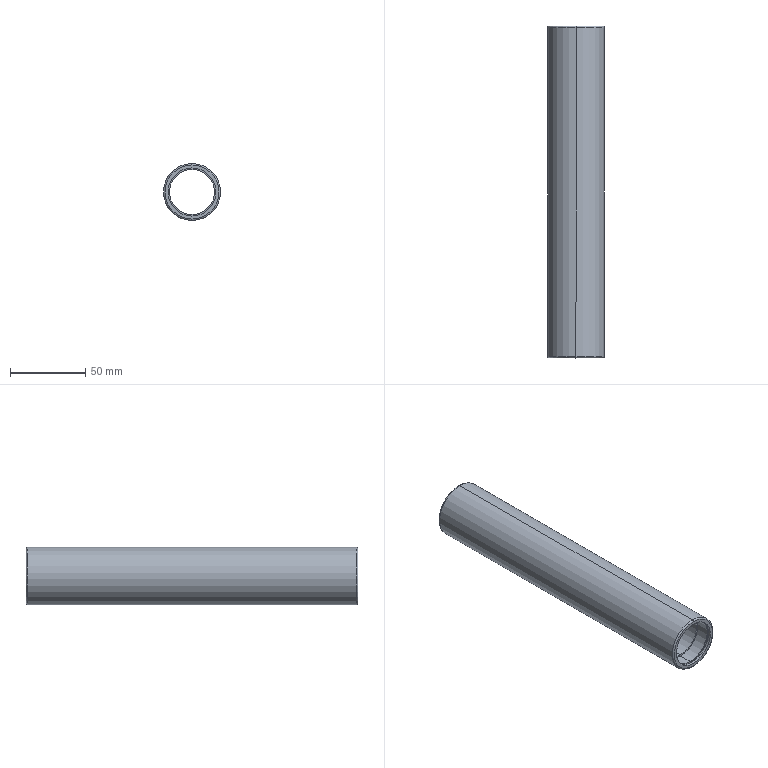Component | SolidWorks | 8TC-A15004-83-00-16_8TC-A15004-80-13A-1 | 1 solid | 28 faces | box 38 x 221 x 38 mm | volume 91799 mm3 | cylinder 16 | plane 8 | torus 4 | commonest cylinder face diameters 32 x8 33.7 x4 38 x2 30 x2 | material #45
build123d program:
from build123d import *

# Parameters (mm, degrees)
FILLET1_R = 1


with BuildPart() as part:
    # Sketch1 → Revolve1 (revolve)
    with BuildSketch(Plane(origin=(0, 0, 0), x_dir=(1, 0, 0), z_dir=(0, 1, 0)), mode=Mode.PRIVATE) as revolve1_sk:
        Polygon((98.5, 15), (-98.5, 15), (-98.5, 16), (-107.5, 16), (-107.5, 16.85), (-108.85, 16.85), (-108.85, 16), (-110.5, 16), (-110.5, 19), (110.5, 19), (110.5, 16), (108.85, 16), (108.85, 16.85), (107.5, 16.85), (107.5, 16), (98.5, 16), align=None)
    revolve(revolve1_sk.sketch.rotate(Axis((-29.776, 0, 0), (1, 0, 0)), 180), axis=Axis((-29.776, 0, 0), (1, 0, 0)))

    # Fillet1
    fillet1_edges = [part.edges().sort_by_distance(p)[0] for p in [
        (-110.5, 0, -19),
        (110.5, 0, -19),
    ]]
    fillet(fillet1_edges, radius=FILLET1_R)


solid = part.part

# Placed as in the assembly
solid = solid.moved(Location((40, 130, 60), (0, 0, 90)))
STEP:
#1=COLOUR_RGB('',0.7922,0.8196,0.9333);
#2=FILL_AREA_STYLE_COLOUR('',#1);
#3=FILL_AREA_STYLE('',(#2));
#4=SURFACE_STYLE_FILL_AREA(#3);
#5=SURFACE_SIDE_STYLE('',(#4));
#6=SURFACE_STYLE_USAGE(.BOTH.,#5);
#7=PRESENTATION_STYLE_ASSIGNMENT((#6));
#8=CARTESIAN_POINT('',(1.575,0.7677,3.071));
#9=VERTEX_POINT('',#8);
#10=CARTESIAN_POINT('',(1.575,0.7677,1.654));
#11=VERTEX_POINT('',#10);
#12=CARTESIAN_POINT('',(1.575,0.7677,2.362));
#13=DIRECTION('',(-0.,-1.,0.));
#14=DIRECTION('',(0.,0.,-1.));
#15=AXIS2_PLACEMENT_3D('',#12,#13,#14);
#16=CIRCLE('',#15,0.7087);
#17=EDGE_CURVE('',#9,#11,#16,.T.);
#18=ORIENTED_EDGE('',*,*,#17,.F.);
#19=CARTESIAN_POINT('',(1.575,0.8071,3.11));
#20=VERTEX_POINT('',#19);
#21=CARTESIAN_POINT('',(1.575,0.8071,3.071));
#22=DIRECTION('',(-1.,0.,-0.));
#23=DIRECTION('',(0.,-1.,0.));
#24=AXIS2_PLACEMENT_3D('',#21,#22,#23);
#25=CIRCLE('',#24,0.03937);
#26=EDGE_CURVE('',#9,#20,#25,.T.);
#27=ORIENTED_EDGE('',*,*,#26,.T.);
#28=CARTESIAN_POINT('',(1.575,0.8071,1.614));
#29=VERTEX_POINT('',#28);
#30=CARTESIAN_POINT('',(1.575,0.8071,2.362));
#31=DIRECTION('',(0.,1.,0.));
#32=DIRECTION('',(0.,0.,-1.));
#33=AXIS2_PLACEMENT_3D('',#30,#31,#32);
#34=CIRCLE('',#33,0.748);
#35=EDGE_CURVE('',#29,#20,#34,.T.);
#36=ORIENTED_EDGE('',*,*,#35,.F.);
#37=CARTESIAN_POINT('',(1.575,0.8071,1.654));
#38=DIRECTION('',(1.,-0.,0.));
#39=DIRECTION('',(0.,1.,0.));
#40=AXIS2_PLACEMENT_3D('',#37,#38,#39);
#41=CIRCLE('',#40,0.03937);
#42=EDGE_CURVE('',#11,#29,#41,.T.);
#43=ORIENTED_EDGE('',*,*,#42,.F.);
#44=EDGE_LOOP('',(#18,#27,#36,#43));
#45=FACE_OUTER_BOUND('',#44,.T.);
#46=CARTESIAN_POINT('',(1.575,0.8071,2.362));
#47=DIRECTION('',(0.,1.,0.));
#48=DIRECTION('',(0.,0.,-1.));
#49=AXIS2_PLACEMENT_3D('',#46,#47,#48);
#50=TOROIDAL_SURFACE('',#49,0.7087,0.03937);
#51=ADVANCED_FACE('',(#45),#50,.T.);
#52=CARTESIAN_POINT('',(1.575,9.469,1.654));
#53=VERTEX_POINT('',#52);
#54=CARTESIAN_POINT('',(1.575,9.469,3.071));
#55=VERTEX_POINT('',#54);
#56=CARTESIAN_POINT('',(1.575,9.469,2.362));
#57=DIRECTION('',(0.,1.,0.));
#58=DIRECTION('',(0.,0.,1.));
#59=AXIS2_PLACEMENT_3D('',#56,#57,#58);
#60=CIRCLE('',#59,0.7087);
#61=EDGE_CURVE('',#53,#55,#60,.T.);
#62=ORIENTED_EDGE('',*,*,#61,.F.);
#63=CARTESIAN_POINT('',(1.575,9.429,1.614));
#64=VERTEX_POINT('',#63);
#65=CARTESIAN_POINT('',(1.575,9.429,1.654));
#66=DIRECTION('',(-1.,0.,0.));
#67=DIRECTION('',(0.,-1.,0.));
#68=AXIS2_PLACEMENT_3D('',#65,#66,#67);
#69=CIRCLE('',#68,0.03937);
#70=EDGE_CURVE('',#53,#64,#69,.T.);
#71=ORIENTED_EDGE('',*,*,#70,.T.);
#72=CARTESIAN_POINT('',(1.575,9.429,3.11));
#73=VERTEX_POINT('',#72);
#74=CARTESIAN_POINT('',(1.575,9.429,2.362));
#75=DIRECTION('',(-0.,-1.,0.));
#76=DIRECTION('',(0.,0.,1.));
#77=AXIS2_PLACEMENT_3D('',#74,#75,#76);
#78=CIRCLE('',#77,0.748);
#79=EDGE_CURVE('',#73,#64,#78,.T.);
#80=ORIENTED_EDGE('',*,*,#79,.F.);
#81=CARTESIAN_POINT('',(1.575,9.429,3.071));
#82=DIRECTION('',(1.,-0.,0.));
#83=DIRECTION('',(0.,1.,0.));
#84=AXIS2_PLACEMENT_3D('',#81,#82,#83);
#85=CIRCLE('',#84,0.03937);
#86=EDGE_CURVE('',#55,#73,#85,.T.);
#87=ORIENTED_EDGE('',*,*,#86,.F.);
#88=EDGE_LOOP('',(#62,#71,#80,#87));
#89=FACE_OUTER_BOUND('',#88,.T.);
#90=CARTESIAN_POINT('',(1.575,9.429,2.362));
#91=DIRECTION('',(-0.,-1.,0.));
#92=DIRECTION('',(0.,0.,1.));
#93=AXIS2_PLACEMENT_3D('',#90,#91,#92);
#94=TOROIDAL_SURFACE('',#93,0.7087,0.03937);
#95=ADVANCED_FACE('',(#89),#94,.T.);
#96=CARTESIAN_POINT('',(1.575,1.24,1.732));
#97=VERTEX_POINT('',#96);
#98=CARTESIAN_POINT('',(1.575,1.24,2.992));
#99=VERTEX_POINT('',#98);
#100=CARTESIAN_POINT('',(1.575,1.24,2.362));
#101=DIRECTION('',(-0.,-1.,0.));
#102=DIRECTION('',(0.,0.,1.));
#103=AXIS2_PLACEMENT_3D('',#100,#101,#102);
#104=CIRCLE('',#103,0.6299);
#105=EDGE_CURVE('',#97,#99,#104,.T.);
#106=ORIENTED_EDGE('',*,*,#105,.F.);
#107=CARTESIAN_POINT('',(1.575,0.8858,1.732));
#108=VERTEX_POINT('',#107);
#109=CARTESIAN_POINT('',(1.575,3.946,1.732));
#110=DIRECTION('',(-0.,-1.,0.));
#111=VECTOR('',#110,39.37);
#112=LINE('',#109,#111);
#113=EDGE_CURVE('',#97,#108,#112,.T.);
#114=ORIENTED_EDGE('',*,*,#113,.T.);
#115=CARTESIAN_POINT('',(1.575,0.8858,2.992));
#116=VERTEX_POINT('',#115);
#117=CARTESIAN_POINT('',(1.575,0.8858,2.362));
#118=DIRECTION('',(-0.,-1.,0.));
#119=DIRECTION('',(0.,0.,1.));
#120=AXIS2_PLACEMENT_3D('',#117,#118,#119);
#121=CIRCLE('',#120,0.6299);
#122=EDGE_CURVE('',#108,#116,#121,.T.);
#123=ORIENTED_EDGE('',*,*,#122,.T.);
#124=CARTESIAN_POINT('',(1.575,3.946,2.992));
#125=DIRECTION('',(-0.,-1.,0.));
#126=VECTOR('',#125,39.37);
#127=LINE('',#124,#126);
#128=EDGE_CURVE('',#99,#116,#127,.T.);
#129=ORIENTED_EDGE('',*,*,#128,.F.);
#130=EDGE_LOOP('',(#106,#114,#123,#129));
#131=FACE_OUTER_BOUND('',#130,.T.);
#132=CARTESIAN_POINT('',(1.575,3.946,2.362));
#133=DIRECTION('',(-0.,-1.,0.));
#134=DIRECTION('',(0.,0.,1.));
#135=AXIS2_PLACEMENT_3D('',#132,#133,#134);
#136=CYLINDRICAL_SURFACE('',#135,0.6299);
#137=ADVANCED_FACE('',(#131),#136,.F.);
#138=CARTESIAN_POINT('',(1.575,0.8858,1.699));
#139=VERTEX_POINT('',#138);
#140=CARTESIAN_POINT('',(1.575,0.8858,3.026));
#141=VERTEX_POINT('',#140);
#142=CARTESIAN_POINT('',(1.575,0.8858,2.362));
#143=DIRECTION('',(-0.,-1.,0.));
#144=DIRECTION('',(0.,0.,1.));
#145=AXIS2_PLACEMENT_3D('',#142,#143,#144);
#146=CIRCLE('',#145,0.6634);
#147=EDGE_CURVE('',#139,#141,#146,.T.);
#148=ORIENTED_EDGE('',*,*,#147,.F.);
#149=CARTESIAN_POINT('',(1.575,0.8327,1.699));
#150=VERTEX_POINT('',#149);
#151=CARTESIAN_POINT('',(1.575,3.946,1.699));
#152=DIRECTION('',(-0.,-1.,0.));
#153=VECTOR('',#152,39.37);
#154=LINE('',#151,#153);
#155=EDGE_CURVE('',#139,#150,#154,.T.);
#156=ORIENTED_EDGE('',*,*,#155,.T.);
#157=CARTESIAN_POINT('',(1.575,0.8327,3.026));
#158=VERTEX_POINT('',#157);
#159=CARTESIAN_POINT('',(1.575,0.8327,2.362));
#160=DIRECTION('',(-0.,-1.,0.));
#161=DIRECTION('',(0.,0.,1.));
#162=AXIS2_PLACEMENT_3D('',#159,#160,#161);
#163=CIRCLE('',#162,0.6634);
#164=EDGE_CURVE('',#150,#158,#163,.T.);
#165=ORIENTED_EDGE('',*,*,#164,.T.);
#166=CARTESIAN_POINT('',(1.575,3.946,3.026));
#167=DIRECTION('',(-0.,-1.,0.));
#168=VECTOR('',#167,39.37);
#169=LINE('',#166,#168);
#170=EDGE_CURVE('',#141,#158,#169,.T.);
#171=ORIENTED_EDGE('',*,*,#170,.F.);
#172=EDGE_LOOP('',(#148,#156,#165,#171));
#173=FACE_OUTER_BOUND('',#172,.T.);
#174=CARTESIAN_POINT('',(1.575,3.946,2.362));
#175=DIRECTION('',(-0.,-1.,0.));
#176=DIRECTION('',(0.,0.,1.));
#177=AXIS2_PLACEMENT_3D('',#174,#175,#176);
#178=CYLINDRICAL_SURFACE('',#177,0.6634);
#179=ADVANCED_FACE('',(#173),#178,.F.);
#180=CARTESIAN_POINT('',(1.575,0.8327,1.732));
#181=VERTEX_POINT('',#180);
#182=CARTESIAN_POINT('',(1.575,0.8327,2.992));
#183=VERTEX_POINT('',#182);
#184=CARTESIAN_POINT('',(1.575,0.8327,2.362));
#185=DIRECTION('',(-0.,-1.,0.));
#186=DIRECTION('',(0.,0.,1.));
#187=AXIS2_PLACEMENT_3D('',#184,#185,#186);
#188=CIRCLE('',#187,0.6299);
#189=EDGE_CURVE('',#181,#183,#188,.T.);
#190=ORIENTED_EDGE('',*,*,#189,.F.);
#191=CARTESIAN_POINT('',(1.575,0.7677,1.732));
#192=VERTEX_POINT('',#191);
#193=CARTESIAN_POINT('',(1.575,3.946,1.732));
#194=DIRECTION('',(-0.,-1.,0.));
#195=VECTOR('',#194,39.37);
#196=LINE('',#193,#195);
#197=EDGE_CURVE('',#181,#192,#196,.T.);
#198=ORIENTED_EDGE('',*,*,#197,.T.);
#199=CARTESIAN_POINT('',(1.575,0.7677,2.992));
#200=VERTEX_POINT('',#199);
#201=CARTESIAN_POINT('',(1.575,0.7677,2.362));
#202=DIRECTION('',(-0.,-1.,0.));
#203=DIRECTION('',(0.,0.,1.));
#204=AXIS2_PLACEMENT_3D('',#201,#202,#203);
#205=CIRCLE('',#204,0.6299);
#206=EDGE_CURVE('',#192,#200,#205,.T.);
#207=ORIENTED_EDGE('',*,*,#206,.T.);
#208=CARTESIAN_POINT('',(1.575,3.946,2.992));
#209=DIRECTION('',(-0.,-1.,0.));
#210=VECTOR('',#209,39.37);
#211=LINE('',#208,#210);
#212=EDGE_CURVE('',#183,#200,#211,.T.);
#213=ORIENTED_EDGE('',*,*,#212,.F.);
#214=EDGE_LOOP('',(#190,#198,#207,#213));
#215=FACE_OUTER_BOUND('',#214,.T.);
#216=CARTESIAN_POINT('',(1.575,3.946,2.362));
#217=DIRECTION('',(-0.,-1.,0.));
#218=DIRECTION('',(0.,0.,1.));
#219=AXIS2_PLACEMENT_3D('',#216,#217,#218);
#220=CYLINDRICAL_SURFACE('',#219,0.6299);
#221=ADVANCED_FACE('',(#215),#220,.F.);
#222=ORIENTED_EDGE('',*,*,#79,.T.);
#223=CARTESIAN_POINT('',(1.575,3.946,1.614));
#224=DIRECTION('',(-0.,-1.,0.));
#225=VECTOR('',#224,39.37);
#226=LINE('',#223,#225);
#227=EDGE_CURVE('',#64,#29,#226,.T.);
#228=ORIENTED_EDGE('',*,*,#227,.T.);
#229=ORIENTED_EDGE('',*,*,#35,.T.);
#230=CARTESIAN_POINT('',(1.575,3.946,3.11));
#231=DIRECTION('',(-0.,-1.,0.));
#232=VECTOR('',#231,39.37);
#233=LINE('',#230,#232);
#234=EDGE_CURVE('',#73,#20,#233,.T.);
#235=ORIENTED_EDGE('',*,*,#234,.F.);
#236=EDGE_LOOP('',(#222,#228,#229,#235));
#237=FACE_OUTER_BOUND('',#236,.T.);
#238=CARTESIAN_POINT('',(1.575,3.946,2.362));
#239=DIRECTION('',(-0.,-1.,0.));
#240=DIRECTION('',(0.,0.,1.));
#241=AXIS2_PLACEMENT_3D('',#238,#239,#240);
#242=CYLINDRICAL_SURFACE('',#241,0.748);
#243=ADVANCED_FACE('',(#237),#242,.T.);
#244=CARTESIAN_POINT('',(1.575,9.469,1.732));
#245=VERTEX_POINT('',#244);
#246=CARTESIAN_POINT('',(1.575,9.469,2.992));
#247=VERTEX_POINT('',#246);
#248=CARTESIAN_POINT('',(1.575,9.469,2.362));
#249=DIRECTION('',(-0.,-1.,0.));
#250=DIRECTION('',(0.,0.,1.));
#251=AXIS2_PLACEMENT_3D('',#248,#249,#250);
#252=CIRCLE('',#251,0.6299);
#253=EDGE_CURVE('',#245,#247,#252,.T.);
#254=ORIENTED_EDGE('',*,*,#253,.F.);
#255=CARTESIAN_POINT('',(1.575,9.404,1.732));
#256=VERTEX_POINT('',#255);
#257=CARTESIAN_POINT('',(1.575,3.946,1.732));
#258=DIRECTION('',(-0.,-1.,0.));
#259=VECTOR('',#258,39.37);
#260=LINE('',#257,#259);
#261=EDGE_CURVE('',#245,#256,#260,.T.);
#262=ORIENTED_EDGE('',*,*,#261,.T.);
#263=CARTESIAN_POINT('',(1.575,9.404,2.992));
#264=VERTEX_POINT('',#263);
#265=CARTESIAN_POINT('',(1.575,9.404,2.362));
#266=DIRECTION('',(-0.,-1.,0.));
#267=DIRECTION('',(0.,0.,1.));
#268=AXIS2_PLACEMENT_3D('',#265,#266,#267);
#269=CIRCLE('',#268,0.6299);
#270=EDGE_CURVE('',#256,#264,#269,.T.);
#271=ORIENTED_EDGE('',*,*,#270,.T.);
#272=CARTESIAN_POINT('',(1.575,3.946,2.992));
#273=DIRECTION('',(-0.,-1.,0.));
#274=VECTOR('',#273,39.37);
#275=LINE('',#272,#274);
#276=EDGE_CURVE('',#247,#264,#275,.T.);
#277=ORIENTED_EDGE('',*,*,#276,.F.);
#278=EDGE_LOOP('',(#254,#262,#271,#277));
#279=FACE_OUTER_BOUND('',#278,.T.);
#280=CARTESIAN_POINT('',(1.575,3.946,2.362));
#281=DIRECTION('',(-0.,-1.,0.));
#282=DIRECTION('',(0.,0.,1.));
#283=AXIS2_PLACEMENT_3D('',#280,#281,#282);
#284=CYLINDRICAL_SURFACE('',#283,0.6299);
#285=ADVANCED_FACE('',(#279),#284,.F.);
#286=CARTESIAN_POINT('',(1.575,9.404,1.699));
#287=VERTEX_POINT('',#286);
#288=CARTESIAN_POINT('',(1.575,9.404,3.026));
#289=VERTEX_POINT('',#288);
#290=CARTESIAN_POINT('',(1.575,9.404,2.362));
#291=DIRECTION('',(-0.,-1.,0.));
#292=DIRECTION('',(0.,0.,1.));
#293=AXIS2_PLACEMENT_3D('',#290,#291,#292);
#294=CIRCLE('',#293,0.6634);
#295=EDGE_CURVE('',#287,#289,#294,.T.);
#296=ORIENTED_EDGE('',*,*,#295,.F.);
#297=CARTESIAN_POINT('',(1.575,9.35,1.699));
#298=VERTEX_POINT('',#297);
#299=CARTESIAN_POINT('',(1.575,3.946,1.699));
#300=DIRECTION('',(-0.,-1.,0.));
#301=VECTOR('',#300,39.37);
#302=LINE('',#299,#301);
#303=EDGE_CURVE('',#287,#298,#302,.T.);
#304=ORIENTED_EDGE('',*,*,#303,.T.);
#305=CARTESIAN_POINT('',(1.575,9.35,3.026));
#306=VERTEX_POINT('',#305);
#307=CARTESIAN_POINT('',(1.575,9.35,2.362));
#308=DIRECTION('',(-0.,-1.,0.));
#309=DIRECTION('',(0.,0.,1.));
#310=AXIS2_PLACEMENT_3D('',#307,#308,#309);
#311=CIRCLE('',#310,0.6634);
#312=EDGE_CURVE('',#298,#306,#311,.T.);
#313=ORIENTED_EDGE('',*,*,#312,.T.);
#314=CARTESIAN_POINT('',(1.575,3.946,3.026));
#315=DIRECTION('',(-0.,-1.,0.));
#316=VECTOR('',#315,39.37);
#317=LINE('',#314,#316);
#318=EDGE_CURVE('',#289,#306,#317,.T.);
#319=ORIENTED_EDGE('',*,*,#318,.F.);
#320=EDGE_LOOP('',(#296,#304,#313,#319));
#321=FACE_OUTER_BOUND('',#320,.T.);
#322=CARTESIAN_POINT('',(1.575,3.946,2.362));
#323=DIRECTION('',(-0.,-1.,0.));
#324=DIRECTION('',(0.,0.,1.));
#325=AXIS2_PLACEMENT_3D('',#322,#323,#324);
#326=CYLINDRICAL_SURFACE('',#325,0.6634);
#327=ADVANCED_FACE('',(#321),#326,.F.);
#328=CARTESIAN_POINT('',(1.575,9.35,1.732));
#329=VERTEX_POINT('',#328);
#330=CARTESIAN_POINT('',(1.575,9.35,2.992));
#331=VERTEX_POINT('',#330);
#332=CARTESIAN_POINT('',(1.575,9.35,2.362));
#333=DIRECTION('',(-0.,-1.,0.));
#334=DIRECTION('',(0.,0.,1.));
#335=AXIS2_PLACEMENT_3D('',#332,#333,#334);
#336=CIRCLE('',#335,0.6299);
#337=EDGE_CURVE('',#329,#331,#336,.T.);
#338=ORIENTED_EDGE('',*,*,#337,.F.);
#339=CARTESIAN_POINT('',(1.575,8.996,1.732));
#340=VERTEX_POINT('',#339);
#341=CARTESIAN_POINT('',(1.575,3.946,1.732));
#342=DIRECTION('',(-0.,-1.,0.));
#343=VECTOR('',#342,39.37);
#344=LINE('',#341,#343);
#345=EDGE_CURVE('',#329,#340,#344,.T.);
#346=ORIENTED_EDGE('',*,*,#345,.T.);
#347=CARTESIAN_POINT('',(1.575,8.996,2.992));
#348=VERTEX_POINT('',#347);
#349=CARTESIAN_POINT('',(1.575,8.996,2.362));
#350=DIRECTION('',(-0.,-1.,0.));
#351=DIRECTION('',(0.,0.,1.));
#352=AXIS2_PLACEMENT_3D('',#349,#350,#351);
#353=CIRCLE('',#352,0.6299);
#354=EDGE_CURVE('',#340,#348,#353,.T.);
#355=ORIENTED_EDGE('',*,*,#354,.T.);
#356=CARTESIAN_POINT('',(1.575,3.946,2.992));
#357=DIRECTION('',(-0.,-1.,0.));
#358=VECTOR('',#357,39.37);
#359=LINE('',#356,#358);
#360=EDGE_CURVE('',#331,#348,#359,.T.);
#361=ORIENTED_EDGE('',*,*,#360,.F.);
#362=EDGE_LOOP('',(#338,#346,#355,#361));
#363=FACE_OUTER_BOUND('',#362,.T.);
#364=CARTESIAN_POINT('',(1.575,3.946,2.362));
#365=DIRECTION('',(-0.,-1.,0.));
#366=DIRECTION('',(0.,0.,1.));
#367=AXIS2_PLACEMENT_3D('',#364,#365,#366);
#368=CYLINDRICAL_SURFACE('',#367,0.6299);
#369=ADVANCED_FACE('',(#363),#368,.F.);
#370=CARTESIAN_POINT('',(1.575,8.996,1.772));
#371=VERTEX_POINT('',#370);
#372=CARTESIAN_POINT('',(1.575,8.996,2.953));
#373=VERTEX_POINT('',#372);
#374=CARTESIAN_POINT('',(1.575,8.996,2.362));
#375=DIRECTION('',(-0.,-1.,0.));
#376=DIRECTION('',(0.,0.,1.));
#377=AXIS2_PLACEMENT_3D('',#374,#375,#376);
#378=CIRCLE('',#377,0.5906);
#379=EDGE_CURVE('',#371,#373,#378,.T.);
#380=ORIENTED_EDGE('',*,*,#379,.F.);
#381=CARTESIAN_POINT('',(1.575,1.24,1.772));
#382=VERTEX_POINT('',#381);
#383=CARTESIAN_POINT('',(1.575,3.946,1.772));
#384=DIRECTION('',(-0.,-1.,0.));
#385=VECTOR('',#384,39.37);
#386=LINE('',#383,#385);
#387=EDGE_CURVE('',#371,#382,#386,.T.);
#388=ORIENTED_EDGE('',*,*,#387,.T.);
#389=CARTESIAN_POINT('',(1.575,1.24,2.953));
#390=VERTEX_POINT('',#389);
#391=CARTESIAN_POINT('',(1.575,1.24,2.362));
#392=DIRECTION('',(-0.,-1.,0.));
#393=DIRECTION('',(0.,0.,1.));
#394=AXIS2_PLACEMENT_3D('',#391,#392,#393);
#395=CIRCLE('',#394,0.5906);
#396=EDGE_CURVE('',#382,#390,#395,.T.);
#397=ORIENTED_EDGE('',*,*,#396,.T.);
#398=CARTESIAN_POINT('',(1.575,3.946,2.953));
#399=DIRECTION('',(-0.,-1.,0.));
#400=VECTOR('',#399,39.37);
#401=LINE('',#398,#400);
#402=EDGE_CURVE('',#373,#390,#401,.T.);
#403=ORIENTED_EDGE('',*,*,#402,.F.);
#404=EDGE_LOOP('',(#380,#388,#397,#403));
#405=FACE_OUTER_BOUND('',#404,.T.);
#406=CARTESIAN_POINT('',(1.575,3.946,2.362));
#407=DIRECTION('',(-0.,-1.,0.));
#408=DIRECTION('',(0.,0.,1.));
#409=AXIS2_PLACEMENT_3D('',#406,#407,#408);
#410=CYLINDRICAL_SURFACE('',#409,0.5906);
#411=ADVANCED_FACE('',(#405),#410,.F.);
#412=CARTESIAN_POINT('',(1.575,1.24,2.362));
#413=DIRECTION('',(-0.,-1.,0.));
#414=DIRECTION('',(0.,0.,1.));
#415=AXIS2_PLACEMENT_3D('',#412,#413,#414);
#416=CIRCLE('',#415,0.5906);
#417=EDGE_CURVE('',#390,#382,#416,.T.);
#418=ORIENTED_EDGE('',*,*,#417,.F.);
#419=ORIENTED_EDGE('',*,*,#396,.F.);
#420=EDGE_LOOP('',(#418,#419));
#421=FACE_BOUND('',#420,.T.);
#422=CARTESIAN_POINT('',(1.575,1.24,2.362));
#423=DIRECTION('',(-0.,-1.,0.));
#424=DIRECTION('',(0.,0.,1.));
#425=AXIS2_PLACEMENT_3D('',#422,#423,#424);
#426=CIRCLE('',#425,0.6299);
#427=EDGE_CURVE('',#99,#97,#426,.T.);
#428=ORIENTED_EDGE('',*,*,#427,.T.);
#429=ORIENTED_EDGE('',*,*,#105,.T.);
#430=EDGE_LOOP('',(#428,#429));
#431=FACE_OUTER_BOUND('',#430,.T.);
#432=CARTESIAN_POINT('',(1.575,1.24,1.772));
#433=DIRECTION('',(0.,1.,0.));
#434=DIRECTION('',(0.,0.,-1.));
#435=AXIS2_PLACEMENT_3D('',#432,#433,#434);
#436=PLANE('',#435);
#437=ADVANCED_FACE('',(#421,#431),#436,.F.);
#438=ORIENTED_EDGE('',*,*,#387,.F.);
#439=CARTESIAN_POINT('',(1.575,8.996,2.362));
#440=DIRECTION('',(-0.,-1.,0.));
#441=DIRECTION('',(0.,0.,1.));
#442=AXIS2_PLACEMENT_3D('',#439,#440,#441);
#443=CIRCLE('',#442,0.5906);
#444=EDGE_CURVE('',#373,#371,#443,.T.);
#445=ORIENTED_EDGE('',*,*,#444,.F.);
#446=ORIENTED_EDGE('',*,*,#402,.T.);
#447=ORIENTED_EDGE('',*,*,#417,.T.);
#448=EDGE_LOOP('',(#438,#445,#446,#447));
#449=FACE_OUTER_BOUND('',#448,.T.);
#450=CARTESIAN_POINT('',(1.575,3.946,2.362));
#451=DIRECTION('',(-0.,-1.,0.));
#452=DIRECTION('',(0.,0.,1.));
#453=AXIS2_PLACEMENT_3D('',#450,#451,#452);
#454=CYLINDRICAL_SURFACE('',#453,0.5906);
#455=ADVANCED_FACE('',(#449),#454,.F.);
#456=CARTESIAN_POINT('',(1.575,8.996,2.362));
#457=DIRECTION('',(-0.,-1.,0.));
#458=DIRECTION('',(0.,0.,1.));
#459=AXIS2_PLACEMENT_3D('',#456,#457,#458);
#460=CIRCLE('',#459,0.6299);
#461=EDGE_CURVE('',#348,#340,#460,.T.);
#462=ORIENTED_EDGE('',*,*,#461,.F.);
#463=ORIENTED_EDGE('',*,*,#354,.F.);
#464=EDGE_LOOP('',(#462,#463));
#465=FACE_OUTER_BOUND('',#464,.T.);
#466=ORIENTED_EDGE('',*,*,#444,.T.);
#467=ORIENTED_EDGE('',*,*,#379,.T.);
#468=EDGE_LOOP('',(#466,#467));
#469=FACE_BOUND('',#468,.T.);
#470=CARTESIAN_POINT('',(1.575,8.996,1.772));
#471=DIRECTION('',(-0.,-1.,0.));
#472=DIRECTION('',(0.,0.,1.));
#473=AXIS2_PLACEMENT_3D('',#470,#471,#472);
#474=PLANE('',#473);
#475=ADVANCED_FACE('',(#465,#469),#474,.F.);
#476=ORIENTED_EDGE('',*,*,#345,.F.);
#477=CARTESIAN_POINT('',(1.575,9.35,2.362));
#478=DIRECTION('',(-0.,-1.,0.));
#479=DIRECTION('',(0.,0.,1.));
#480=AXIS2_PLACEMENT_3D('',#477,#478,#479);
#481=CIRCLE('',#480,0.6299);
#482=EDGE_CURVE('',#331,#329,#481,.T.);
#483=ORIENTED_EDGE('',*,*,#482,.F.);
#484=ORIENTED_EDGE('',*,*,#360,.T.);
#485=ORIENTED_EDGE('',*,*,#461,.T.);
#486=EDGE_LOOP('',(#476,#483,#484,#485));
#487=FACE_OUTER_BOUND('',#486,.T.);
#488=CARTESIAN_POINT('',(1.575,3.946,2.362));
#489=DIRECTION('',(-0.,-1.,0.));
#490=DIRECTION('',(0.,0.,1.));
#491=AXIS2_PLACEMENT_3D('',#488,#489,#490);
#492=CYLINDRICAL_SURFACE('',#491,0.6299);
#493=ADVANCED_FACE('',(#487),#492,.F.);
#494=CARTESIAN_POINT('',(1.575,9.35,2.362));
#495=DIRECTION('',(-0.,-1.,0.));
#496=DIRECTION('',(0.,0.,1.));
#497=AXIS2_PLACEMENT_3D('',#494,#495,#496);
#498=CIRCLE('',#497,0.6634);
#499=EDGE_CURVE('',#306,#298,#498,.T.);
#500=ORIENTED_EDGE('',*,*,#499,.F.);
#501=ORIENTED_EDGE('',*,*,#312,.F.);
#502=EDGE_LOOP('',(#500,#501));
#503=FACE_OUTER_BOUND('',#502,.T.);
#504=ORIENTED_EDGE('',*,*,#482,.T.);
#505=ORIENTED_EDGE('',*,*,#337,.T.);
#506=EDGE_LOOP('',(#504,#505));
#507=FACE_BOUND('',#506,.T.);
#508=CARTESIAN_POINT('',(1.575,9.35,1.732));
#509=DIRECTION('',(-0.,-1.,0.));
#510=DIRECTION('',(0.,0.,1.));
#511=AXIS2_PLACEMENT_3D('',#508,#509,#510);
#512=PLANE('',#511);
#513=ADVANCED_FACE('',(#503,#507),#512,.F.);
#514=ORIENTED_EDGE('',*,*,#303,.F.);
#515=CARTESIAN_POINT('',(1.575,9.404,2.362));
#516=DIRECTION('',(-0.,-1.,0.));
#517=DIRECTION('',(0.,0.,1.));
#518=AXIS2_PLACEMENT_3D('',#515,#516,#517);
#519=CIRCLE('',#518,0.6634);
#520=EDGE_CURVE('',#289,#287,#519,.T.);
#521=ORIENTED_EDGE('',*,*,#520,.F.);
#522=ORIENTED_EDGE('',*,*,#318,.T.);
#523=ORIENTED_EDGE('',*,*,#499,.T.);
#524=EDGE_LOOP('',(#514,#521,#522,#523));
#525=FACE_OUTER_BOUND('',#524,.T.);
#526=CARTESIAN_POINT('',(1.575,3.946,2.362));
#527=DIRECTION('',(-0.,-1.,0.));
#528=DIRECTION('',(0.,0.,1.));
#529=AXIS2_PLACEMENT_3D('',#526,#527,#528);
#530=CYLINDRICAL_SURFACE('',#529,0.6634);
#531=ADVANCED_FACE('',(#525),#530,.F.);
#532=CARTESIAN_POINT('',(1.575,9.404,2.362));
#533=DIRECTION('',(-0.,-1.,0.));
#534=DIRECTION('',(0.,0.,1.));
#535=AXIS2_PLACEMENT_3D('',#532,#533,#534);
#536=CIRCLE('',#535,0.6299);
#537=EDGE_CURVE('',#264,#256,#536,.T.);
#538=ORIENTED_EDGE('',*,*,#537,.F.);
#539=ORIENTED_EDGE('',*,*,#270,.F.);
#540=EDGE_LOOP('',(#538,#539));
#541=FACE_BOUND('',#540,.T.);
#542=ORIENTED_EDGE('',*,*,#520,.T.);
#543=ORIENTED_EDGE('',*,*,#295,.T.);
#544=EDGE_LOOP('',(#542,#543));
#545=FACE_OUTER_BOUND('',#544,.T.);
#546=CARTESIAN_POINT('',(1.575,9.404,1.699));
#547=DIRECTION('',(0.,1.,0.));
#548=DIRECTION('',(0.,0.,-1.));
#549=AXIS2_PLACEMENT_3D('',#546,#547,#548);
#550=PLANE('',#549);
#551=ADVANCED_FACE('',(#541,#545),#550,.F.);
#552=ORIENTED_EDGE('',*,*,#261,.F.);
#553=CARTESIAN_POINT('',(1.575,9.469,2.362));
#554=DIRECTION('',(-0.,-1.,0.));
#555=DIRECTION('',(0.,0.,1.));
#556=AXIS2_PLACEMENT_3D('',#553,#554,#555);
#557=CIRCLE('',#556,0.6299);
#558=EDGE_CURVE('',#247,#245,#557,.T.);
#559=ORIENTED_EDGE('',*,*,#558,.F.);
#560=ORIENTED_EDGE('',*,*,#276,.T.);
#561=ORIENTED_EDGE('',*,*,#537,.T.);
#562=EDGE_LOOP('',(#552,#559,#560,#561));
#563=FACE_OUTER_BOUND('',#562,.T.);
#564=CARTESIAN_POINT('',(1.575,3.946,2.362));
#565=DIRECTION('',(-0.,-1.,0.));
#566=DIRECTION('',(0.,0.,1.));
#567=AXIS2_PLACEMENT_3D('',#564,#565,#566);
#568=CYLINDRICAL_SURFACE('',#567,0.6299);
#569=ADVANCED_FACE('',(#563),#568,.F.);
#570=CARTESIAN_POINT('',(1.575,9.469,2.362));
#571=DIRECTION('',(0.,1.,0.));
#572=DIRECTION('',(0.,0.,1.));
#573=AXIS2_PLACEMENT_3D('',#570,#571,#572);
#574=CIRCLE('',#573,0.7087);
#575=EDGE_CURVE('',#55,#53,#574,.T.);
#576=ORIENTED_EDGE('',*,*,#575,.T.);
#577=ORIENTED_EDGE('',*,*,#61,.T.);
#578=EDGE_LOOP('',(#576,#577));
#579=FACE_OUTER_BOUND('',#578,.T.);
#580=ORIENTED_EDGE('',*,*,#558,.T.);
#581=ORIENTED_EDGE('',*,*,#253,.T.);
#582=EDGE_LOOP('',(#580,#581));
#583=FACE_BOUND('',#582,.T.);
#584=CARTESIAN_POINT('',(1.575,9.469,1.732));
#585=DIRECTION('',(-0.,-1.,0.));
#586=DIRECTION('',(0.,0.,1.));
#587=AXIS2_PLACEMENT_3D('',#584,#585,#586);
#588=PLANE('',#587);
#589=ADVANCED_FACE('',(#579,#583),#588,.F.);
#590=ORIENTED_EDGE('',*,*,#227,.F.);
#591=CARTESIAN_POINT('',(1.575,9.429,2.362));
#592=DIRECTION('',(-0.,-1.,0.));
#593=DIRECTION('',(0.,0.,1.));
#594=AXIS2_PLACEMENT_3D('',#591,#592,#593);
#595=CIRCLE('',#594,0.748);
#596=EDGE_CURVE('',#64,#73,#595,.T.);
#597=ORIENTED_EDGE('',*,*,#596,.T.);
#598=ORIENTED_EDGE('',*,*,#234,.T.);
#599=CARTESIAN_POINT('',(1.575,0.8071,2.362));
#600=DIRECTION('',(0.,1.,0.));
#601=DIRECTION('',(0.,0.,-1.));
#602=AXIS2_PLACEMENT_3D('',#599,#600,#601);
#603=CIRCLE('',#602,0.748);
#604=EDGE_CURVE('',#20,#29,#603,.T.);
#605=ORIENTED_EDGE('',*,*,#604,.T.);
#606=EDGE_LOOP('',(#590,#597,#598,#605));
#607=FACE_OUTER_BOUND('',#606,.T.);
#608=CARTESIAN_POINT('',(1.575,3.946,2.362));
#609=DIRECTION('',(-0.,-1.,0.));
#610=DIRECTION('',(0.,0.,1.));
#611=AXIS2_PLACEMENT_3D('',#608,#609,#610);
#612=CYLINDRICAL_SURFACE('',#611,0.748);
#613=ADVANCED_FACE('',(#607),#612,.T.);
#614=CARTESIAN_POINT('',(1.575,0.7677,2.362));
#615=DIRECTION('',(-0.,-1.,0.));
#616=DIRECTION('',(0.,0.,-1.));
#617=AXIS2_PLACEMENT_3D('',#614,#615,#616);
#618=CIRCLE('',#617,0.7087);
#619=EDGE_CURVE('',#11,#9,#618,.T.);
#620=ORIENTED_EDGE('',*,*,#619,.T.);
#621=ORIENTED_EDGE('',*,*,#17,.T.);
#622=EDGE_LOOP('',(#620,#621));
#623=FACE_OUTER_BOUND('',#622,.T.);
#624=CARTESIAN_POINT('',(1.575,0.7677,2.362));
#625=DIRECTION('',(-0.,-1.,0.));
#626=DIRECTION('',(0.,0.,1.));
#627=AXIS2_PLACEMENT_3D('',#624,#625,#626);
#628=CIRCLE('',#627,0.6299);
#629=EDGE_CURVE('',#200,#192,#628,.T.);
#630=ORIENTED_EDGE('',*,*,#629,.F.);
#631=ORIENTED_EDGE('',*,*,#206,.F.);
#632=EDGE_LOOP('',(#630,#631));
#633=FACE_BOUND('',#632,.T.);
#634=CARTESIAN_POINT('',(1.575,0.7677,1.732));
#635=DIRECTION('',(0.,1.,0.));
#636=DIRECTION('',(0.,0.,-1.));
#637=AXIS2_PLACEMENT_3D('',#634,#635,#636);
#638=PLANE('',#637);
#639=ADVANCED_FACE('',(#623,#633),#638,.F.);
#640=ORIENTED_EDGE('',*,*,#197,.F.);
#641=CARTESIAN_POINT('',(1.575,0.8327,2.362));
#642=DIRECTION('',(-0.,-1.,0.));
#643=DIRECTION('',(0.,0.,1.));
#644=AXIS2_PLACEMENT_3D('',#641,#642,#643);
#645=CIRCLE('',#644,0.6299);
#646=EDGE_CURVE('',#183,#181,#645,.T.);
#647=ORIENTED_EDGE('',*,*,#646,.F.);
#648=ORIENTED_EDGE('',*,*,#212,.T.);
#649=ORIENTED_EDGE('',*,*,#629,.T.);
#650=EDGE_LOOP('',(#640,#647,#648,#649));
#651=FACE_OUTER_BOUND('',#650,.T.);
#652=CARTESIAN_POINT('',(1.575,3.946,2.362));
#653=DIRECTION('',(-0.,-1.,0.));
#654=DIRECTION('',(0.,0.,1.));
#655=AXIS2_PLACEMENT_3D('',#652,#653,#654);
#656=CYLINDRICAL_SURFACE('',#655,0.6299);
#657=ADVANCED_FACE('',(#651),#656,.F.);
#658=CARTESIAN_POINT('',(1.575,0.8327,2.362));
#659=DIRECTION('',(-0.,-1.,0.));
#660=DIRECTION('',(0.,0.,1.));
#661=AXIS2_PLACEMENT_3D('',#658,#659,#660);
#662=CIRCLE('',#661,0.6634);
#663=EDGE_CURVE('',#158,#150,#662,.T.);
#664=ORIENTED_EDGE('',*,*,#663,.F.);
#665=ORIENTED_EDGE('',*,*,#164,.F.);
#666=EDGE_LOOP('',(#664,#665));
#667=FACE_OUTER_BOUND('',#666,.T.);
#668=ORIENTED_EDGE('',*,*,#646,.T.);
#669=ORIENTED_EDGE('',*,*,#189,.T.);
#670=EDGE_LOOP('',(#668,#669));
#671=FACE_BOUND('',#670,.T.);
#672=CARTESIAN_POINT('',(1.575,0.8327,1.699));
#673=DIRECTION('',(-0.,-1.,0.));
#674=DIRECTION('',(0.,0.,1.));
#675=AXIS2_PLACEMENT_3D('',#672,#673,#674);
#676=PLANE('',#675);
#677=ADVANCED_FACE('',(#667,#671),#676,.F.);
#678=ORIENTED_EDGE('',*,*,#155,.F.);
#679=CARTESIAN_POINT('',(1.575,0.8858,2.362));
#680=DIRECTION('',(-0.,-1.,0.));
#681=DIRECTION('',(0.,0.,1.));
#682=AXIS2_PLACEMENT_3D('',#679,#680,#681);
#683=CIRCLE('',#682,0.6634);
#684=EDGE_CURVE('',#141,#139,#683,.T.);
#685=ORIENTED_EDGE('',*,*,#684,.F.);
#686=ORIENTED_EDGE('',*,*,#170,.T.);
#687=ORIENTED_EDGE('',*,*,#663,.T.);
#688=EDGE_LOOP('',(#678,#685,#686,#687));
#689=FACE_OUTER_BOUND('',#688,.T.);
#690=CARTESIAN_POINT('',(1.575,3.946,2.362));
#691=DIRECTION('',(-0.,-1.,0.));
#692=DIRECTION('',(0.,0.,1.));
#693=AXIS2_PLACEMENT_3D('',#690,#691,#692);
#694=CYLINDRICAL_SURFACE('',#693,0.6634);
#695=ADVANCED_FACE('',(#689),#694,.F.);
#696=CARTESIAN_POINT('',(1.575,0.8858,2.362));
#697=DIRECTION('',(-0.,-1.,0.));
#698=DIRECTION('',(0.,0.,1.));
#699=AXIS2_PLACEMENT_3D('',#696,#697,#698);
#700=CIRCLE('',#699,0.6299);
#701=EDGE_CURVE('',#116,#108,#700,.T.);
#702=ORIENTED_EDGE('',*,*,#701,.F.);
#703=ORIENTED_EDGE('',*,*,#122,.F.);
#704=EDGE_LOOP('',(#702,#703));
#705=FACE_BOUND('',#704,.T.);
#706=ORIENTED_EDGE('',*,*,#684,.T.);
#707=ORIENTED_EDGE('',*,*,#147,.T.);
#708=EDGE_LOOP('',(#706,#707));
#709=FACE_OUTER_BOUND('',#708,.T.);
#710=CARTESIAN_POINT('',(1.575,0.8858,1.732));
#711=DIRECTION('',(0.,1.,0.));
#712=DIRECTION('',(0.,0.,-1.));
#713=AXIS2_PLACEMENT_3D('',#710,#711,#712);
#714=PLANE('',#713);
#715=ADVANCED_FACE('',(#705,#709),#714,.F.);
#716=ORIENTED_EDGE('',*,*,#113,.F.);
#717=ORIENTED_EDGE('',*,*,#427,.F.);
#718=ORIENTED_EDGE('',*,*,#128,.T.);
#719=ORIENTED_EDGE('',*,*,#701,.T.);
#720=EDGE_LOOP('',(#716,#717,#718,#719));
#721=FACE_OUTER_BOUND('',#720,.T.);
#722=CARTESIAN_POINT('',(1.575,3.946,2.362));
#723=DIRECTION('',(-0.,-1.,0.));
#724=DIRECTION('',(0.,0.,1.));
#725=AXIS2_PLACEMENT_3D('',#722,#723,#724);
#726=CYLINDRICAL_SURFACE('',#725,0.6299);
#727=ADVANCED_FACE('',(#721),#726,.F.);
#728=ORIENTED_EDGE('',*,*,#70,.F.);
#729=ORIENTED_EDGE('',*,*,#575,.F.);
#730=ORIENTED_EDGE('',*,*,#86,.T.);
#731=ORIENTED_EDGE('',*,*,#596,.F.);
#732=EDGE_LOOP('',(#728,#729,#730,#731));
#733=FACE_OUTER_BOUND('',#732,.T.);
#734=CARTESIAN_POINT('',(1.575,9.429,2.362));
#735=DIRECTION('',(-0.,-1.,0.));
#736=DIRECTION('',(0.,0.,1.));
#737=AXIS2_PLACEMENT_3D('',#734,#735,#736);
#738=TOROIDAL_SURFACE('',#737,0.7087,0.03937);
#739=ADVANCED_FACE('',(#733),#738,.T.);
#740=ORIENTED_EDGE('',*,*,#26,.F.);
#741=ORIENTED_EDGE('',*,*,#619,.F.);
#742=ORIENTED_EDGE('',*,*,#42,.T.);
#743=ORIENTED_EDGE('',*,*,#604,.F.);
#744=EDGE_LOOP('',(#740,#741,#742,#743));
#745=FACE_OUTER_BOUND('',#744,.T.);
#746=CARTESIAN_POINT('',(1.575,0.8071,2.362));
#747=DIRECTION('',(0.,1.,0.));
#748=DIRECTION('',(0.,0.,-1.));
#749=AXIS2_PLACEMENT_3D('',#746,#747,#748);
#750=TOROIDAL_SURFACE('',#749,0.7087,0.03937);
#751=ADVANCED_FACE('',(#745),#750,.T.);
#752=CLOSED_SHELL('',(#51,#95,#137,#179,#221,#243,#285,#327,#369,#411,#437,#455,#475,#493,#513,#531,#551,#569,#589,#613,#639,#657,#677,#695,#715,#727,#739,#751));
#753=MANIFOLD_SOLID_BREP('',#752);
#754=STYLED_ITEM('',(#7),#753);
#755=(LENGTH_UNIT()NAMED_UNIT(*)SI_UNIT($,.METRE.));
#756=LENGTH_MEASURE_WITH_UNIT(LENGTH_MEASURE(0.0254),#755);
#757=DIMENSIONAL_EXPONENTS(1.,0.,0.,0.,0.,0.,0.);
#758=(CONVERSION_BASED_UNIT('',#756)LENGTH_UNIT()NAMED_UNIT(#757));
#759=UNCERTAINTY_MEASURE_WITH_UNIT(LENGTH_MEASURE(0.00001),#758,'','');
#760=(NAMED_UNIT(*)PLANE_ANGLE_UNIT()SI_UNIT($,.RADIAN.));
#761=(NAMED_UNIT(*)SI_UNIT($,.STERADIAN.)SOLID_ANGLE_UNIT());
#762=(GEOMETRIC_REPRESENTATION_CONTEXT(3)GLOBAL_UNCERTAINTY_ASSIGNED_CONTEXT((#759))GLOBAL_UNIT_ASSIGNED_CONTEXT((#758,#760,#761))REPRESENTATION_CONTEXT('',''));
#763=MECHANICAL_DESIGN_GEOMETRIC_PRESENTATION_REPRESENTATION('',(#754),#762);
#764=CARTESIAN_POINT('',(0.,0.,0.));
#765=DIRECTION('',(0.,0.,1.));
#766=DIRECTION('',(1.,0.,0.));
#767=AXIS2_PLACEMENT_3D('',#764,#765,#766);
#768=(LENGTH_UNIT()NAMED_UNIT(*)SI_UNIT($,.METRE.));
#769=LENGTH_MEASURE_WITH_UNIT(LENGTH_MEASURE(0.0254),#768);
#770=DIMENSIONAL_EXPONENTS(1.,0.,0.,0.,0.,0.,0.);
#771=(CONVERSION_BASED_UNIT('',#769)LENGTH_UNIT()NAMED_UNIT(#770));
#772=UNCERTAINTY_MEASURE_WITH_UNIT(LENGTH_MEASURE(0.00001),#771,'','');
#773=(NAMED_UNIT(*)PLANE_ANGLE_UNIT()SI_UNIT($,.RADIAN.));
#774=(NAMED_UNIT(*)SI_UNIT($,.STERADIAN.)SOLID_ANGLE_UNIT());
#775=(GEOMETRIC_REPRESENTATION_CONTEXT(3)GLOBAL_UNCERTAINTY_ASSIGNED_CONTEXT((#772))GLOBAL_UNIT_ASSIGNED_CONTEXT((#771,#773,#774))REPRESENTATION_CONTEXT('',''));
#776=ADVANCED_BREP_SHAPE_REPRESENTATION('',(#753,#767),#775);
#777=PRESENTATION_LAYER_ASSIGNMENT('','',(#754));